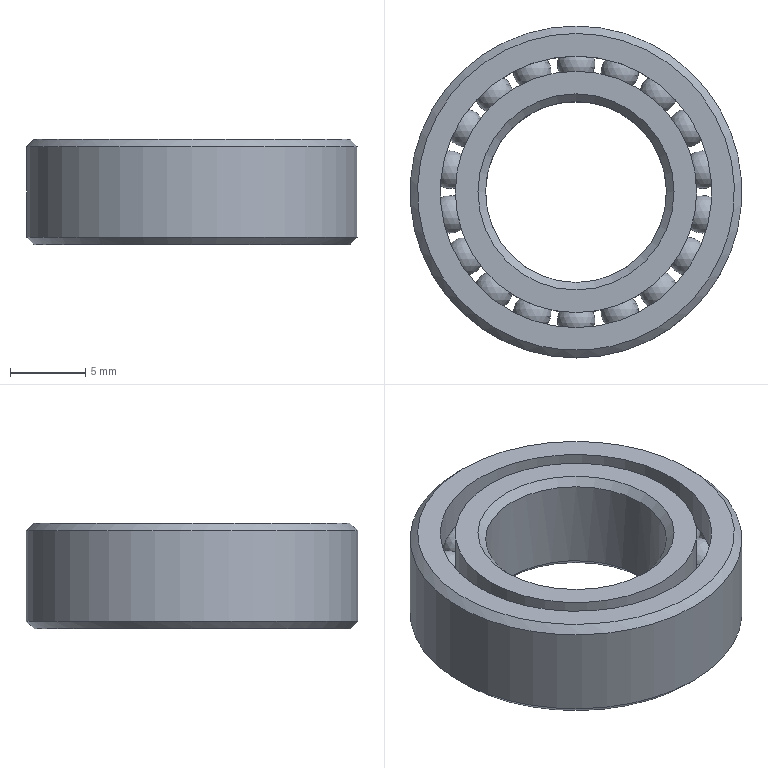Component | NX | BEARING | 20 solids | 34 faces | volume 1484 mm3 | sphere 18 | cylinder 6 | plane 4 | cone 4 | torus 2 | commonest cylinder face diameters 16 x2 18 x2 12 x1 22 x1